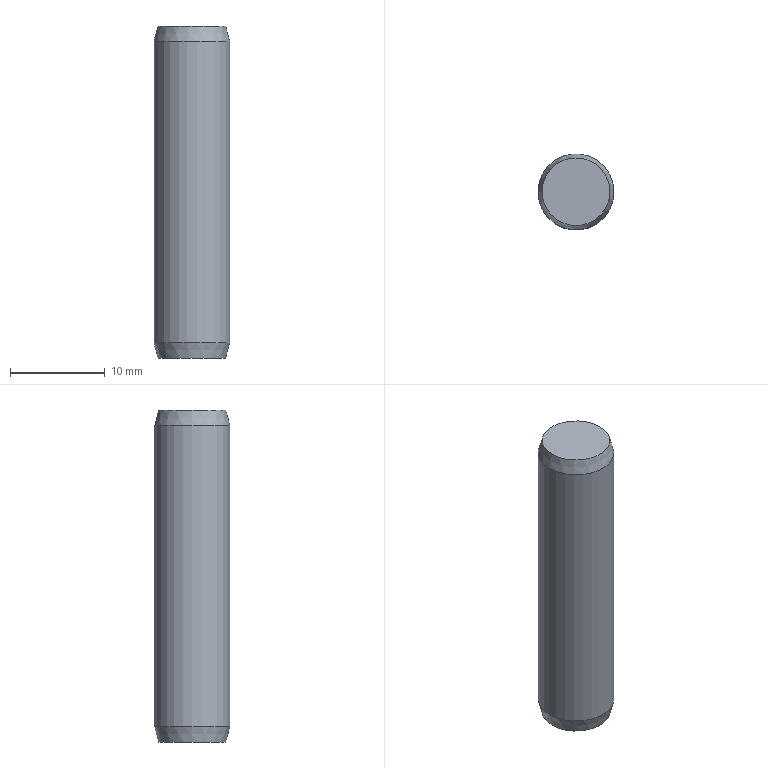Component | NX | GB-T119_1-2000_8X35 | 1 solid | 5 faces | box 8 x 8 x 35 mm | volume 1743 mm3 | plane 2 | cone 2 | cylinder 1 | commonest cylinder face diameters 8 x1
STEP:
#1=CARTESIAN_POINT('',(0.,0.,0.));
#2=DIRECTION('',(0.,0.,1.));
#3=DIRECTION('',(1.,0.,0.));
#4=AXIS2_PLACEMENT_3D('',#1,#2,#3);
#5=CARTESIAN_POINT('',(-63.571,20.5,18.));
#6=VERTEX_POINT('',#5);
#7=CARTESIAN_POINT('',(-60.,20.5,18.));
#8=DIRECTION('',(0.,0.,-1.));
#9=DIRECTION('',(-1.,0.,0.));
#10=AXIS2_PLACEMENT_3D('',#7,#8,#9);
#11=CIRCLE('',#10,3.571);
#12=CARTESIAN_POINT('',(-60.,20.5,18.));
#13=DIRECTION('',(0.,0.,-1.));
#14=DIRECTION('',(-1.,0.,0.));
#15=AXIS2_PLACEMENT_3D('',#12,#13,#14);
#16=PLANE('',#15);
#17=CARTESIAN_POINT('',(0.,0.));
#18=DIRECTION('',(1.,0.));
#19=AXIS2_PLACEMENT_2D('',#17,#18);
#20=CIRCLE('',#19,3.571);
#21=(GEOMETRIC_REPRESENTATION_CONTEXT(2)PARAMETRIC_REPRESENTATION_CONTEXT()REPRESENTATION_CONTEXT('',''));
#22=DEFINITIONAL_REPRESENTATION('',(#20),#21);
#23=PCURVE('',#16,#22);
#24=CARTESIAN_POINT('',(-60.,20.5,18.));
#25=DIRECTION('',(0.,0.,1.));
#26=DIRECTION('',(1.,0.,0.));
#27=AXIS2_PLACEMENT_3D('',#24,#25,#26);
#28=CONICAL_SURFACE('',#27,3.571,0.2618);
#29=CARTESIAN_POINT('',(9.425,0.));
#30=DIRECTION('',(-1.,0.));
#31=VECTOR('',#30,1.);
#32=LINE('',#29,#31);
#33=(GEOMETRIC_REPRESENTATION_CONTEXT(2)PARAMETRIC_REPRESENTATION_CONTEXT()REPRESENTATION_CONTEXT('',''));
#34=DEFINITIONAL_REPRESENTATION('',(#32),#33);
#35=PCURVE('',#28,#34);
#36=SURFACE_CURVE('',#11,(#23,#35),.PCURVE_S1.);
#37=EDGE_CURVE('',#6,#6,#36,.T.);
#38=ORIENTED_EDGE('',*,*,#37,.T.);
#39=EDGE_LOOP('',(#38));
#40=FACE_BOUND('',#39,.T.);
#41=ADVANCED_FACE('',(#40),#16,.T.);
#42=CARTESIAN_POINT('',(-64.,20.5,19.6));
#43=VERTEX_POINT('',#42);
#44=CARTESIAN_POINT('',(-60.,20.5,19.6));
#45=DIRECTION('',(0.,0.,-1.));
#46=DIRECTION('',(-1.,0.,0.));
#47=AXIS2_PLACEMENT_3D('',#44,#45,#46);
#48=CIRCLE('',#47,4.);
#49=CARTESIAN_POINT('',(9.425,1.6));
#50=DIRECTION('',(-1.,0.));
#51=VECTOR('',#50,1.);
#52=LINE('',#49,#51);
#53=(GEOMETRIC_REPRESENTATION_CONTEXT(2)PARAMETRIC_REPRESENTATION_CONTEXT()REPRESENTATION_CONTEXT('',''));
#54=DEFINITIONAL_REPRESENTATION('',(#52),#53);
#55=PCURVE('',#28,#54);
#56=CARTESIAN_POINT('',(-60.,20.5,53.));
#57=DIRECTION('',(0.,0.,-1.));
#58=DIRECTION('',(-1.,0.,0.));
#59=AXIS2_PLACEMENT_3D('',#56,#57,#58);
#60=CYLINDRICAL_SURFACE('',#59,4.);
#61=CARTESIAN_POINT('',(0.,33.4));
#62=DIRECTION('',(1.,0.));
#63=VECTOR('',#62,1.);
#64=LINE('',#61,#63);
#65=(GEOMETRIC_REPRESENTATION_CONTEXT(2)PARAMETRIC_REPRESENTATION_CONTEXT()REPRESENTATION_CONTEXT('',''));
#66=DEFINITIONAL_REPRESENTATION('',(#64),#65);
#67=PCURVE('',#60,#66);
#68=SURFACE_CURVE('',#48,(#55,#67),.PCURVE_S1.);
#69=EDGE_CURVE('',#43,#43,#68,.T.);
#70=ORIENTED_EDGE('',*,*,#69,.T.);
#71=CARTESIAN_POINT('',(-63.571,20.5,18.));
#72=CARTESIAN_POINT('',(-64.,20.5,19.6));
#73=B_SPLINE_CURVE_WITH_KNOTS('',1,(#71,#72),.UNSPECIFIED.,.F.,.F.,(2,2),(0.,1.656),.PIECEWISE_BEZIER_KNOTS.);
#74=CARTESIAN_POINT('',(3.142,0.));
#75=DIRECTION('',(0.,1.));
#76=VECTOR('',#75,1.);
#77=LINE('',#74,#76);
#78=(GEOMETRIC_REPRESENTATION_CONTEXT(2)PARAMETRIC_REPRESENTATION_CONTEXT()REPRESENTATION_CONTEXT('',''));
#79=DEFINITIONAL_REPRESENTATION('',(#77),#78);
#80=PCURVE('',#28,#79);
#81=CARTESIAN_POINT('',(9.425,0.));
#82=DIRECTION('',(0.,1.));
#83=VECTOR('',#82,1.);
#84=LINE('',#81,#83);
#85=(GEOMETRIC_REPRESENTATION_CONTEXT(2)PARAMETRIC_REPRESENTATION_CONTEXT()REPRESENTATION_CONTEXT('',''));
#86=DEFINITIONAL_REPRESENTATION('',(#84),#85);
#87=PCURVE('',#28,#86);
#88=SEAM_CURVE('',#73,(#80,#87),.PCURVE_S1.);
#89=EDGE_CURVE('',#6,#43,#88,.T.);
#90=ORIENTED_EDGE('',*,*,#89,.F.);
#91=ORIENTED_EDGE('',*,*,#37,.F.);
#92=ORIENTED_EDGE('',*,*,#89,.T.);
#93=EDGE_LOOP('',(#70,#90,#91,#92));
#94=FACE_BOUND('',#93,.T.);
#95=ADVANCED_FACE('',(#94),#28,.T.);
#96=CARTESIAN_POINT('',(-64.,20.5,51.4));
#97=VERTEX_POINT('',#96);
#98=CARTESIAN_POINT('',(-60.,20.5,51.4));
#99=DIRECTION('',(0.,0.,-1.));
#100=DIRECTION('',(-1.,0.,0.));
#101=AXIS2_PLACEMENT_3D('',#98,#99,#100);
#102=CIRCLE('',#101,4.);
#103=CARTESIAN_POINT('',(0.,1.6));
#104=DIRECTION('',(1.,0.));
#105=VECTOR('',#104,1.);
#106=LINE('',#103,#105);
#107=(GEOMETRIC_REPRESENTATION_CONTEXT(2)PARAMETRIC_REPRESENTATION_CONTEXT()REPRESENTATION_CONTEXT('',''));
#108=DEFINITIONAL_REPRESENTATION('',(#106),#107);
#109=PCURVE('',#60,#108);
#110=CARTESIAN_POINT('',(-60.,20.5,51.4));
#111=DIRECTION('',(0.,0.,-1.));
#112=DIRECTION('',(-1.,0.,0.));
#113=AXIS2_PLACEMENT_3D('',#110,#111,#112);
#114=CONICAL_SURFACE('',#113,4.,0.2618);
#115=CARTESIAN_POINT('',(0.,0.));
#116=DIRECTION('',(1.,0.));
#117=VECTOR('',#116,1.);
#118=LINE('',#115,#117);
#119=(GEOMETRIC_REPRESENTATION_CONTEXT(2)PARAMETRIC_REPRESENTATION_CONTEXT()REPRESENTATION_CONTEXT('',''));
#120=DEFINITIONAL_REPRESENTATION('',(#118),#119);
#121=PCURVE('',#114,#120);
#122=SURFACE_CURVE('',#102,(#109,#121),.PCURVE_S1.);
#123=EDGE_CURVE('',#97,#97,#122,.T.);
#124=ORIENTED_EDGE('',*,*,#123,.T.);
#125=CARTESIAN_POINT('',(-64.,20.5,51.4));
#126=CARTESIAN_POINT('',(-64.,20.5,19.6));
#127=B_SPLINE_CURVE_WITH_KNOTS('',1,(#125,#126),.UNSPECIFIED.,.F.,.F.,(2,2),(1.6,33.4),.PIECEWISE_BEZIER_KNOTS.);
#128=CARTESIAN_POINT('',(6.283,0.));
#129=DIRECTION('',(0.,1.));
#130=VECTOR('',#129,1.);
#131=LINE('',#128,#130);
#132=(GEOMETRIC_REPRESENTATION_CONTEXT(2)PARAMETRIC_REPRESENTATION_CONTEXT()REPRESENTATION_CONTEXT('',''));
#133=DEFINITIONAL_REPRESENTATION('',(#131),#132);
#134=PCURVE('',#60,#133);
#135=CARTESIAN_POINT('',(0.,0.));
#136=DIRECTION('',(0.,1.));
#137=VECTOR('',#136,1.);
#138=LINE('',#135,#137);
#139=(GEOMETRIC_REPRESENTATION_CONTEXT(2)PARAMETRIC_REPRESENTATION_CONTEXT()REPRESENTATION_CONTEXT('',''));
#140=DEFINITIONAL_REPRESENTATION('',(#138),#139);
#141=PCURVE('',#60,#140);
#142=SEAM_CURVE('',#127,(#134,#141),.PCURVE_S1.);
#143=EDGE_CURVE('',#97,#43,#142,.T.);
#144=ORIENTED_EDGE('',*,*,#143,.T.);
#145=ORIENTED_EDGE('',*,*,#69,.F.);
#146=ORIENTED_EDGE('',*,*,#143,.F.);
#147=EDGE_LOOP('',(#124,#144,#145,#146));
#148=FACE_BOUND('',#147,.T.);
#149=ADVANCED_FACE('',(#148),#60,.T.);
#150=CARTESIAN_POINT('',(-63.571,20.5,53.));
#151=VERTEX_POINT('',#150);
#152=CARTESIAN_POINT('',(-60.,20.5,53.));
#153=DIRECTION('',(0.,0.,-1.));
#154=DIRECTION('',(-1.,0.,0.));
#155=AXIS2_PLACEMENT_3D('',#152,#153,#154);
#156=CIRCLE('',#155,3.571);
#157=CARTESIAN_POINT('',(0.,-1.6));
#158=DIRECTION('',(1.,0.));
#159=VECTOR('',#158,1.);
#160=LINE('',#157,#159);
#161=(GEOMETRIC_REPRESENTATION_CONTEXT(2)PARAMETRIC_REPRESENTATION_CONTEXT()REPRESENTATION_CONTEXT('',''));
#162=DEFINITIONAL_REPRESENTATION('',(#160),#161);
#163=PCURVE('',#114,#162);
#164=CARTESIAN_POINT('',(-56.429,20.5,53.));
#165=DIRECTION('',(0.,0.,1.));
#166=DIRECTION('',(1.,0.,0.));
#167=AXIS2_PLACEMENT_3D('',#164,#165,#166);
#168=PLANE('',#167);
#169=CARTESIAN_POINT('',(-7.143,0.));
#170=CARTESIAN_POINT('',(-7.143,6.186));
#171=CARTESIAN_POINT('',(-1.786,3.093));
#172=CARTESIAN_POINT('',(3.571,0.));
#173=CARTESIAN_POINT('',(-1.786,-3.093));
#174=CARTESIAN_POINT('',(-7.143,-6.186));
#175=CARTESIAN_POINT('',(-7.143,0.));
#176=(BOUNDED_CURVE()B_SPLINE_CURVE(2,(#169,#170,#171,#172,#173,#174,#175),.UNSPECIFIED.,.T.,.F.)B_SPLINE_CURVE_WITH_KNOTS((1,2,2,2,2,1),(-2.094,0.,2.094,4.189,6.283,8.378),.UNSPECIFIED.)CURVE()GEOMETRIC_REPRESENTATION_ITEM()RATIONAL_B_SPLINE_CURVE((1.,0.5,1.,0.5,1.,0.5,1.))REPRESENTATION_ITEM(''));
#177=(GEOMETRIC_REPRESENTATION_CONTEXT(2)PARAMETRIC_REPRESENTATION_CONTEXT()REPRESENTATION_CONTEXT('',''));
#178=DEFINITIONAL_REPRESENTATION('',(#176),#177);
#179=PCURVE('',#168,#178);
#180=SURFACE_CURVE('',#156,(#163,#179),.PCURVE_S1.);
#181=EDGE_CURVE('',#151,#151,#180,.T.);
#182=ORIENTED_EDGE('',*,*,#181,.T.);
#183=CARTESIAN_POINT('',(-63.571,20.5,53.));
#184=CARTESIAN_POINT('',(-64.,20.5,51.4));
#185=B_SPLINE_CURVE_WITH_KNOTS('',1,(#183,#184),.UNSPECIFIED.,.F.,.F.,(2,2),(-1.656,0.),.PIECEWISE_BEZIER_KNOTS.);
#186=CARTESIAN_POINT('',(6.283,0.));
#187=DIRECTION('',(0.,1.));
#188=VECTOR('',#187,1.);
#189=LINE('',#186,#188);
#190=(GEOMETRIC_REPRESENTATION_CONTEXT(2)PARAMETRIC_REPRESENTATION_CONTEXT()REPRESENTATION_CONTEXT('',''));
#191=DEFINITIONAL_REPRESENTATION('',(#189),#190);
#192=PCURVE('',#114,#191);
#193=CARTESIAN_POINT('',(0.,0.));
#194=DIRECTION('',(0.,1.));
#195=VECTOR('',#194,1.);
#196=LINE('',#193,#195);
#197=(GEOMETRIC_REPRESENTATION_CONTEXT(2)PARAMETRIC_REPRESENTATION_CONTEXT()REPRESENTATION_CONTEXT('',''));
#198=DEFINITIONAL_REPRESENTATION('',(#196),#197);
#199=PCURVE('',#114,#198);
#200=SEAM_CURVE('',#185,(#192,#199),.PCURVE_S1.);
#201=EDGE_CURVE('',#151,#97,#200,.T.);
#202=ORIENTED_EDGE('',*,*,#201,.T.);
#203=ORIENTED_EDGE('',*,*,#123,.F.);
#204=ORIENTED_EDGE('',*,*,#201,.F.);
#205=EDGE_LOOP('',(#182,#202,#203,#204));
#206=FACE_BOUND('',#205,.T.);
#207=ADVANCED_FACE('',(#206),#114,.T.);
#208=ORIENTED_EDGE('',*,*,#181,.F.);
#209=EDGE_LOOP('',(#208));
#210=FACE_BOUND('',#209,.T.);
#211=ADVANCED_FACE('',(#210),#168,.T.);
#212=CLOSED_SHELL('',(#41,#95,#149,#207,#211));
#213=MANIFOLD_SOLID_BREP('',#212);
#214=(LENGTH_UNIT()NAMED_UNIT(*)SI_UNIT(.MILLI.,.METRE.));
#215=UNCERTAINTY_MEASURE_WITH_UNIT(LENGTH_MEASURE(0.00001),#214,'','');
#216=(NAMED_UNIT(*)PLANE_ANGLE_UNIT()SI_UNIT($,.RADIAN.));
#217=(NAMED_UNIT(*)SI_UNIT($,.STERADIAN.)SOLID_ANGLE_UNIT());
#218=(GEOMETRIC_REPRESENTATION_CONTEXT(3)GLOBAL_UNCERTAINTY_ASSIGNED_CONTEXT((#215))GLOBAL_UNIT_ASSIGNED_CONTEXT((#214,#216,#217))REPRESENTATION_CONTEXT('',''));
#219=ADVANCED_BREP_SHAPE_REPRESENTATION('',(#4,#213),#218);